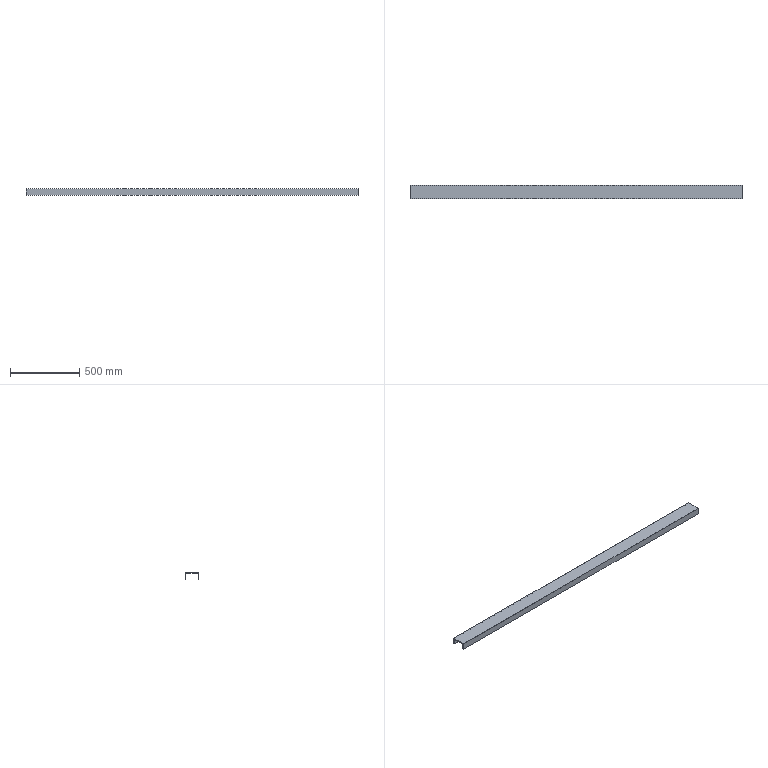Component | SolidWorks | 01FrontBase-1 | 1 solid | 36 faces | box 2400 x 100 x 48 mm | volume 2436384 mm3 | cylinder 26 | plane 10 | commonest cylinder face diameters 10 x26
build123d program:
from build123d import *

# Parameters (mm, degrees)
EXTRUDE_THIN1_DEPTH            = 2400
F_10_0_10_DIAMETER_HOLE1_D     = 10
F_10_0_10_DIAMETER_HOLE1_DEPTH = 5.5


with BuildPart() as part:
    # Sketch1 → Extrude-Thin1 (new body)
    with BuildSketch(Plane.XY):
        Polygon((48, 0), (0, 0), (0, 100), (48, 100), (48, 94.5), (5.5, 94.5), (5.5, 5.5), (48, 5.5), align=None)
    extrude(amount=EXTRUDE_THIN1_DEPTH)

    # 10.0 _10_ Diameter Hole1
    with Locations(Plane(origin=(0, 100, 0), x_dir=(-1, 0, 0), z_dir=(0, 1, 0))):
        with Locations((-18, 18), (-18, 68), (-18, 2332), (-18, 2382), (-18, 200), (-18, 550), (-18, 900), (-18, 2225), (-18, 1875), (-18, 1525), (-18, 1250), (-18, 1380), (-18, 1420)):
            Hole(F_10_0_10_DIAMETER_HOLE1_D / 2, depth=F_10_0_10_DIAMETER_HOLE1_DEPTH)


solid = part.part

# Placed as in the assembly
solid = solid.moved(Location((-123.527, -139.54, 1237.107), (0, 90, 0)))